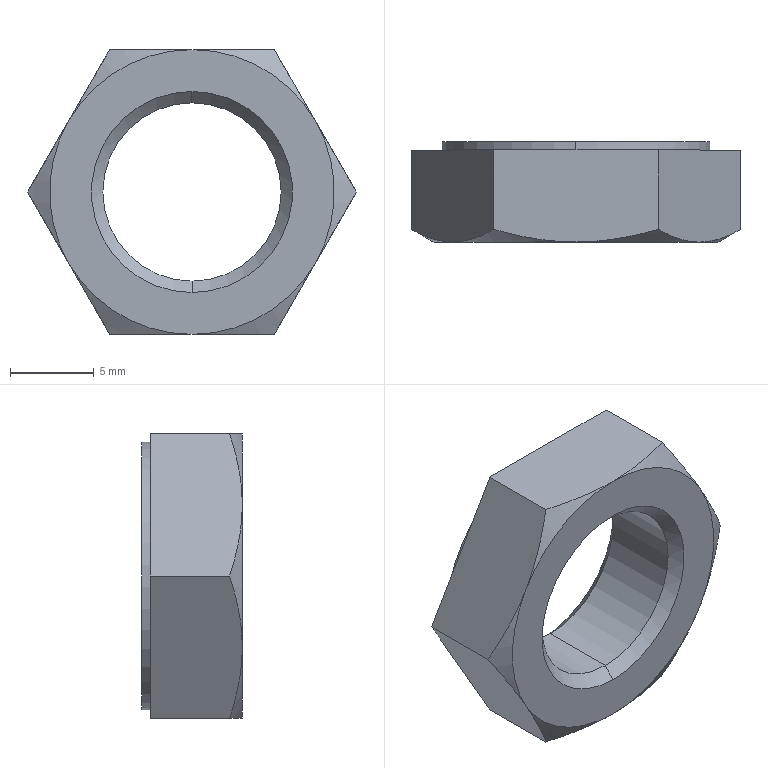Component | SolidWorks | MI-8x60-S-U-M-2(0)-1_MI8-M12x1_25 - Nut-1 | 1 solid | 23 faces | box 19.63 x 6 x 17 mm | volume 922 mm3 | cone 10 | plane 9 | cylinder 4 | commonest cylinder face diameters 10.647 x2 16 x2
build123d program:
from build123d import *

# Parameters (mm, degrees)
SKETCH2_W          = 34
SKETCH2_H          = 34
CUT_EXTRUDE1_DEPTH = 12


with BuildPart() as part:
    # Sketch1 → Revolve1 (revolve)
    with BuildSketch(Plane.XY, mode=Mode.PRIVATE) as revolve1_sk:
        Polygon((0, 0), (0, 8.5), (0.9815, 10.2), (5.5, 10.2), (5.5, 8), (6, 8), (6, 0), align=None)
    revolve(revolve1_sk.sketch.rotate(Axis((6, 0, 0), (-1, 0, 0)), 270), axis=Axis((6, 0, 0), (-1, 0, 0)))

    # Sketch2 → Cut-Extrude1 (cut)
    with BuildSketch(Plane(origin=(0, 0, 0), x_dir=(0, 0, -1), z_dir=(1, 0, 0))):
        Rectangle(SKETCH2_W, SKETCH2_H)
        Polygon((-8.5, 4.907), (-8.5, -4.907), (0, -9.815), (8.5, -4.907), (8.5, 4.907), (0, 9.815), align=None, mode=Mode.SUBTRACT)
    extrude(amount=CUT_EXTRUDE1_DEPTH, mode=Mode.SUBTRACT)

    # Sketch3 → Cut-Revolve1 (revolve, cut)
    with BuildSketch(Plane.XY, mode=Mode.PRIVATE) as cut_revolve1_sk:
        Polygon((0, 0), (0, 6), (0.6765, 5.324), (5.324, 5.324), (6, 6), (6, 0), align=None)
    revolve(cut_revolve1_sk.sketch.rotate(Axis((6, 0, 0), (-1, 0, 0)), 270), axis=Axis((6, 0, 0), (-1, 0, 0)), mode=Mode.SUBTRACT)


solid = part.part

# Placed as in the assembly
solid = solid.moved(Location((-44.181, -56.188, -311.979), (0, 0, 90)))
STEP:
#1=COLOUR_RGB('',0.7922,0.8196,0.9333);
#2=FILL_AREA_STYLE_COLOUR('',#1);
#3=FILL_AREA_STYLE('',(#2));
#4=SURFACE_STYLE_FILL_AREA(#3);
#5=SURFACE_SIDE_STYLE('',(#4));
#6=SURFACE_STYLE_USAGE(.BOTH.,#5);
#7=PRESENTATION_STYLE_ASSIGNMENT((#6));
#8=CARTESIAN_POINT('',(-1.739,-2.003,-12.073));
#9=VERTEX_POINT('',#8);
#10=CARTESIAN_POINT('',(-1.739,-2.003,-12.492));
#11=VERTEX_POINT('',#10);
#12=CARTESIAN_POINT('',(-1.739,-2.003,-12.283));
#13=DIRECTION('',(0.,-1.,0.));
#14=DIRECTION('',(0.,0.,-1.));
#15=AXIS2_PLACEMENT_3D('',#12,#13,#14);
#16=CIRCLE('',#15,0.2096);
#17=EDGE_CURVE('',#9,#11,#16,.T.);
#18=ORIENTED_EDGE('',*,*,#17,.T.);
#19=CARTESIAN_POINT('',(-1.739,-1.976,-12.519));
#20=VERTEX_POINT('',#19);
#21=CARTESIAN_POINT('',(-1.739,-1.976,-12.519));
#22=DIRECTION('',(0.,0.7071,-0.7071));
#23=VECTOR('',#22,39.37);
#24=LINE('',#21,#23);
#25=EDGE_CURVE('',#11,#20,#24,.T.);
#26=ORIENTED_EDGE('',*,*,#25,.T.);
#27=CARTESIAN_POINT('',(-1.739,-1.976,-12.046));
#28=VERTEX_POINT('',#27);
#29=CARTESIAN_POINT('',(-1.739,-1.976,-12.283));
#30=DIRECTION('',(0.,-1.,0.));
#31=DIRECTION('',(0.,0.,-1.));
#32=AXIS2_PLACEMENT_3D('',#29,#30,#31);
#33=CIRCLE('',#32,0.2362);
#34=EDGE_CURVE('',#28,#20,#33,.T.);
#35=ORIENTED_EDGE('',*,*,#34,.F.);
#36=CARTESIAN_POINT('',(-1.739,-1.976,-12.046));
#37=DIRECTION('',(-0.,0.7071,0.7071));
#38=VECTOR('',#37,39.37);
#39=LINE('',#36,#38);
#40=EDGE_CURVE('',#9,#28,#39,.T.);
#41=ORIENTED_EDGE('',*,*,#40,.F.);
#42=EDGE_LOOP('',(#18,#26,#35,#41));
#43=FACE_OUTER_BOUND('',#42,.T.);
#44=CARTESIAN_POINT('',(-1.739,-1.976,-12.283));
#45=DIRECTION('',(-0.,1.,-0.));
#46=DIRECTION('',(-0.,0.,1.));
#47=AXIS2_PLACEMENT_3D('',#44,#45,#46);
#48=CONICAL_SURFACE('',#47,0.2362,0.7854);
#49=ADVANCED_FACE('',(#43),#48,.F.);
#50=ORIENTED_EDGE('',*,*,#17,.F.);
#51=CARTESIAN_POINT('',(-1.739,-2.185,-12.073));
#52=VERTEX_POINT('',#51);
#53=CARTESIAN_POINT('',(-1.739,-1.976,-12.073));
#54=DIRECTION('',(0.,-1.,0.));
#55=VECTOR('',#54,39.37);
#56=LINE('',#53,#55);
#57=EDGE_CURVE('',#9,#52,#56,.T.);
#58=ORIENTED_EDGE('',*,*,#57,.T.);
#59=CARTESIAN_POINT('',(-1.739,-2.185,-12.492));
#60=VERTEX_POINT('',#59);
#61=CARTESIAN_POINT('',(-1.739,-2.185,-12.283));
#62=DIRECTION('',(0.,-1.,0.));
#63=DIRECTION('',(0.,0.,-1.));
#64=AXIS2_PLACEMENT_3D('',#61,#62,#63);
#65=CIRCLE('',#64,0.2096);
#66=EDGE_CURVE('',#52,#60,#65,.T.);
#67=ORIENTED_EDGE('',*,*,#66,.T.);
#68=CARTESIAN_POINT('',(-1.739,-1.976,-12.492));
#69=DIRECTION('',(0.,-1.,0.));
#70=VECTOR('',#69,39.37);
#71=LINE('',#68,#70);
#72=EDGE_CURVE('',#11,#60,#71,.T.);
#73=ORIENTED_EDGE('',*,*,#72,.F.);
#74=EDGE_LOOP('',(#50,#58,#67,#73));
#75=FACE_OUTER_BOUND('',#74,.T.);
#76=CARTESIAN_POINT('',(-1.739,-1.976,-12.283));
#77=DIRECTION('',(0.,-1.,0.));
#78=DIRECTION('',(0.,0.,-1.));
#79=AXIS2_PLACEMENT_3D('',#76,#77,#78);
#80=CYLINDRICAL_SURFACE('',#79,0.2096);
#81=ADVANCED_FACE('',(#75),#80,.F.);
#82=ORIENTED_EDGE('',*,*,#66,.F.);
#83=CARTESIAN_POINT('',(-1.739,-2.212,-12.046));
#84=VERTEX_POINT('',#83);
#85=CARTESIAN_POINT('',(-1.739,-2.185,-12.073));
#86=DIRECTION('',(-0.,-0.7071,0.7071));
#87=VECTOR('',#86,39.37);
#88=LINE('',#85,#87);
#89=EDGE_CURVE('',#52,#84,#88,.T.);
#90=ORIENTED_EDGE('',*,*,#89,.T.);
#91=CARTESIAN_POINT('',(-1.739,-2.212,-12.519));
#92=VERTEX_POINT('',#91);
#93=CARTESIAN_POINT('',(-1.739,-2.212,-12.283));
#94=DIRECTION('',(0.,-1.,0.));
#95=DIRECTION('',(0.,0.,-1.));
#96=AXIS2_PLACEMENT_3D('',#93,#94,#95);
#97=CIRCLE('',#96,0.2362);
#98=EDGE_CURVE('',#84,#92,#97,.T.);
#99=ORIENTED_EDGE('',*,*,#98,.T.);
#100=CARTESIAN_POINT('',(-1.739,-2.185,-12.492));
#101=DIRECTION('',(0.,-0.7071,-0.7071));
#102=VECTOR('',#101,39.37);
#103=LINE('',#100,#102);
#104=EDGE_CURVE('',#60,#92,#103,.T.);
#105=ORIENTED_EDGE('',*,*,#104,.F.);
#106=EDGE_LOOP('',(#82,#90,#99,#105));
#107=FACE_OUTER_BOUND('',#106,.T.);
#108=CARTESIAN_POINT('',(-1.739,-2.185,-12.283));
#109=DIRECTION('',(0.,-1.,0.));
#110=DIRECTION('',(0.,0.,-1.));
#111=AXIS2_PLACEMENT_3D('',#108,#109,#110);
#112=CONICAL_SURFACE('',#111,0.2096,0.7854);
#113=ADVANCED_FACE('',(#107),#112,.F.);
#114=CARTESIAN_POINT('',(-1.739,-1.976,-12.598));
#115=VERTEX_POINT('',#114);
#116=CARTESIAN_POINT('',(-1.739,-1.976,-11.968));
#117=VERTEX_POINT('',#116);
#118=CARTESIAN_POINT('',(-1.739,-1.976,-12.283));
#119=DIRECTION('',(0.,-1.,0.));
#120=DIRECTION('',(0.,0.,-1.));
#121=AXIS2_PLACEMENT_3D('',#118,#119,#120);
#122=CIRCLE('',#121,0.315);
#123=EDGE_CURVE('',#115,#117,#122,.T.);
#124=ORIENTED_EDGE('',*,*,#123,.T.);
#125=CARTESIAN_POINT('',(-1.739,-1.996,-11.968));
#126=VERTEX_POINT('',#125);
#127=CARTESIAN_POINT('',(-1.739,-1.976,-11.968));
#128=DIRECTION('',(0.,-1.,0.));
#129=VECTOR('',#128,39.37);
#130=LINE('',#127,#129);
#131=EDGE_CURVE('',#117,#126,#130,.T.);
#132=ORIENTED_EDGE('',*,*,#131,.T.);
#133=CARTESIAN_POINT('',(-1.739,-1.996,-12.598));
#134=VERTEX_POINT('',#133);
#135=CARTESIAN_POINT('',(-1.739,-1.996,-12.283));
#136=DIRECTION('',(0.,-1.,0.));
#137=DIRECTION('',(0.,0.,-1.));
#138=AXIS2_PLACEMENT_3D('',#135,#136,#137);
#139=CIRCLE('',#138,0.315);
#140=EDGE_CURVE('',#134,#126,#139,.T.);
#141=ORIENTED_EDGE('',*,*,#140,.F.);
#142=CARTESIAN_POINT('',(-1.739,-1.976,-12.598));
#143=DIRECTION('',(0.,-1.,0.));
#144=VECTOR('',#143,39.37);
#145=LINE('',#142,#144);
#146=EDGE_CURVE('',#115,#134,#145,.T.);
#147=ORIENTED_EDGE('',*,*,#146,.F.);
#148=EDGE_LOOP('',(#124,#132,#141,#147));
#149=FACE_OUTER_BOUND('',#148,.T.);
#150=CARTESIAN_POINT('',(-1.739,-1.976,-12.283));
#151=DIRECTION('',(0.,-1.,0.));
#152=DIRECTION('',(0.,0.,-1.));
#153=AXIS2_PLACEMENT_3D('',#150,#151,#152);
#154=CYLINDRICAL_SURFACE('',#153,0.315);
#155=ADVANCED_FACE('',(#149),#154,.T.);
#156=ORIENTED_EDGE('',*,*,#123,.F.);
#157=CARTESIAN_POINT('',(-1.739,-1.976,-12.283));
#158=DIRECTION('',(0.,-1.,0.));
#159=DIRECTION('',(0.,0.,-1.));
#160=AXIS2_PLACEMENT_3D('',#157,#158,#159);
#161=CIRCLE('',#160,0.315);
#162=EDGE_CURVE('',#117,#115,#161,.T.);
#163=ORIENTED_EDGE('',*,*,#162,.F.);
#164=EDGE_LOOP('',(#156,#163));
#165=FACE_OUTER_BOUND('',#164,.T.);
#166=ORIENTED_EDGE('',*,*,#34,.T.);
#167=CARTESIAN_POINT('',(-1.739,-1.976,-12.283));
#168=DIRECTION('',(0.,-1.,0.));
#169=DIRECTION('',(0.,0.,-1.));
#170=AXIS2_PLACEMENT_3D('',#167,#168,#169);
#171=CIRCLE('',#170,0.2362);
#172=EDGE_CURVE('',#20,#28,#171,.T.);
#173=ORIENTED_EDGE('',*,*,#172,.T.);
#174=EDGE_LOOP('',(#166,#173));
#175=FACE_BOUND('',#174,.T.);
#176=CARTESIAN_POINT('',(-1.424,-1.976,-12.283));
#177=DIRECTION('',(0.,-1.,0.));
#178=DIRECTION('',(0.,-0.,-1.));
#179=AXIS2_PLACEMENT_3D('',#176,#177,#178);
#180=PLANE('',#179);
#181=ADVANCED_FACE('',(#165,#175),#180,.F.);
#182=CARTESIAN_POINT('',(-1.739,-2.212,-12.617));
#183=VERTEX_POINT('',#182);
#184=CARTESIAN_POINT('',(-1.45,-2.212,-12.45));
#185=VERTEX_POINT('',#184);
#186=CARTESIAN_POINT('',(-1.739,-2.212,-12.283));
#187=DIRECTION('',(0.,-1.,0.));
#188=DIRECTION('',(0.,0.,-1.));
#189=AXIS2_PLACEMENT_3D('',#186,#187,#188);
#190=CIRCLE('',#189,0.3346);
#191=EDGE_CURVE('',#183,#185,#190,.T.);
#192=ORIENTED_EDGE('',*,*,#191,.T.);
#193=CARTESIAN_POINT('',(-1.45,-2.212,-12.115));
#194=VERTEX_POINT('',#193);
#195=CARTESIAN_POINT('',(-1.739,-2.212,-12.283));
#196=DIRECTION('',(0.,-1.,0.));
#197=DIRECTION('',(0.,0.,-1.));
#198=AXIS2_PLACEMENT_3D('',#195,#196,#197);
#199=CIRCLE('',#198,0.3346);
#200=EDGE_CURVE('',#185,#194,#199,.T.);
#201=ORIENTED_EDGE('',*,*,#200,.T.);
#202=CARTESIAN_POINT('',(-1.739,-2.212,-11.948));
#203=VERTEX_POINT('',#202);
#204=CARTESIAN_POINT('',(-1.739,-2.212,-12.283));
#205=DIRECTION('',(0.,-1.,0.));
#206=DIRECTION('',(0.,0.,-1.));
#207=AXIS2_PLACEMENT_3D('',#204,#205,#206);
#208=CIRCLE('',#207,0.3346);
#209=EDGE_CURVE('',#194,#203,#208,.T.);
#210=ORIENTED_EDGE('',*,*,#209,.T.);
#211=CARTESIAN_POINT('',(-2.029,-2.212,-12.115));
#212=VERTEX_POINT('',#211);
#213=CARTESIAN_POINT('',(-1.739,-2.212,-12.283));
#214=DIRECTION('',(0.,-1.,0.));
#215=DIRECTION('',(0.,0.,-1.));
#216=AXIS2_PLACEMENT_3D('',#213,#214,#215);
#217=CIRCLE('',#216,0.3346);
#218=EDGE_CURVE('',#203,#212,#217,.T.);
#219=ORIENTED_EDGE('',*,*,#218,.T.);
#220=CARTESIAN_POINT('',(-2.029,-2.212,-12.45));
#221=VERTEX_POINT('',#220);
#222=CARTESIAN_POINT('',(-1.739,-2.212,-12.283));
#223=DIRECTION('',(0.,-1.,0.));
#224=DIRECTION('',(0.,0.,-1.));
#225=AXIS2_PLACEMENT_3D('',#222,#223,#224);
#226=CIRCLE('',#225,0.3346);
#227=EDGE_CURVE('',#212,#221,#226,.T.);
#228=ORIENTED_EDGE('',*,*,#227,.T.);
#229=CARTESIAN_POINT('',(-1.739,-2.212,-12.283));
#230=DIRECTION('',(0.,-1.,0.));
#231=DIRECTION('',(0.,0.,-1.));
#232=AXIS2_PLACEMENT_3D('',#229,#230,#231);
#233=CIRCLE('',#232,0.3346);
#234=EDGE_CURVE('',#221,#183,#233,.T.);
#235=ORIENTED_EDGE('',*,*,#234,.T.);
#236=EDGE_LOOP('',(#192,#201,#210,#219,#228,#235));
#237=FACE_OUTER_BOUND('',#236,.T.);
#238=CARTESIAN_POINT('',(-1.739,-2.212,-12.283));
#239=DIRECTION('',(0.,-1.,0.));
#240=DIRECTION('',(0.,0.,-1.));
#241=AXIS2_PLACEMENT_3D('',#238,#239,#240);
#242=CIRCLE('',#241,0.2362);
#243=EDGE_CURVE('',#92,#84,#242,.T.);
#244=ORIENTED_EDGE('',*,*,#243,.F.);
#245=ORIENTED_EDGE('',*,*,#98,.F.);
#246=EDGE_LOOP('',(#244,#245));
#247=FACE_BOUND('',#246,.T.);
#248=CARTESIAN_POINT('',(-1.739,-2.212,-12.283));
#249=DIRECTION('',(-0.,1.,-0.));
#250=DIRECTION('',(-0.,0.,1.));
#251=AXIS2_PLACEMENT_3D('',#248,#249,#250);
#252=PLANE('',#251);
#253=ADVANCED_FACE('',(#237,#247),#252,.F.);
#254=CARTESIAN_POINT('',(-1.546,-1.996,-11.948));
#255=VERTEX_POINT('',#254);
#256=CARTESIAN_POINT('',(-1.353,-1.996,-12.283));
#257=VERTEX_POINT('',#256);
#258=CARTESIAN_POINT('',(-1.349,-1.996,-12.289));
#259=DIRECTION('',(0.5,0.,-0.866));
#260=VECTOR('',#259,39.37);
#261=LINE('',#258,#260);
#262=EDGE_CURVE('',#255,#257,#261,.T.);
#263=ORIENTED_EDGE('',*,*,#262,.T.);
#264=CARTESIAN_POINT('',(-1.546,-1.996,-12.617));
#265=VERTEX_POINT('',#264);
#266=CARTESIAN_POINT('',(-1.349,-1.996,-12.276));
#267=DIRECTION('',(-0.5,-0.,-0.866));
#268=VECTOR('',#267,39.37);
#269=LINE('',#266,#268);
#270=EDGE_CURVE('',#257,#265,#269,.T.);
#271=ORIENTED_EDGE('',*,*,#270,.T.);
#272=CARTESIAN_POINT('',(-1.933,-1.996,-12.617));
#273=VERTEX_POINT('',#272);
#274=CARTESIAN_POINT('',(-1.338,-1.996,-12.617));
#275=DIRECTION('',(-1.,-0.,-0.));
#276=VECTOR('',#275,39.37);
#277=LINE('',#274,#276);
#278=EDGE_CURVE('',#265,#273,#277,.T.);
#279=ORIENTED_EDGE('',*,*,#278,.T.);
#280=CARTESIAN_POINT('',(-2.126,-1.996,-12.283));
#281=VERTEX_POINT('',#280);
#282=CARTESIAN_POINT('',(-1.929,-1.996,-12.624));
#283=DIRECTION('',(-0.5,-0.,0.866));
#284=VECTOR('',#283,39.37);
#285=LINE('',#282,#284);
#286=EDGE_CURVE('',#273,#281,#285,.T.);
#287=ORIENTED_EDGE('',*,*,#286,.T.);
#288=CARTESIAN_POINT('',(-1.933,-1.996,-11.948));
#289=VERTEX_POINT('',#288);
#290=CARTESIAN_POINT('',(-1.929,-1.996,-11.941));
#291=DIRECTION('',(0.5,0.,0.866));
#292=VECTOR('',#291,39.37);
#293=LINE('',#290,#292);
#294=EDGE_CURVE('',#281,#289,#293,.T.);
#295=ORIENTED_EDGE('',*,*,#294,.T.);
#296=CARTESIAN_POINT('',(-1.338,-1.996,-11.948));
#297=DIRECTION('',(1.,0.,0.));
#298=VECTOR('',#297,39.37);
#299=LINE('',#296,#298);
#300=EDGE_CURVE('',#289,#255,#299,.T.);
#301=ORIENTED_EDGE('',*,*,#300,.T.);
#302=EDGE_LOOP('',(#263,#271,#279,#287,#295,#301));
#303=FACE_OUTER_BOUND('',#302,.T.);
#304=ORIENTED_EDGE('',*,*,#140,.T.);
#305=CARTESIAN_POINT('',(-1.739,-1.996,-12.283));
#306=DIRECTION('',(0.,-1.,0.));
#307=DIRECTION('',(0.,0.,-1.));
#308=AXIS2_PLACEMENT_3D('',#305,#306,#307);
#309=CIRCLE('',#308,0.315);
#310=EDGE_CURVE('',#126,#134,#309,.T.);
#311=ORIENTED_EDGE('',*,*,#310,.T.);
#312=EDGE_LOOP('',(#304,#311));
#313=FACE_BOUND('',#312,.T.);
#314=CARTESIAN_POINT('',(-1.338,-1.996,-12.283));
#315=DIRECTION('',(0.,-1.,0.));
#316=DIRECTION('',(0.,-0.,-1.));
#317=AXIS2_PLACEMENT_3D('',#314,#315,#316);
#318=PLANE('',#317);
#319=ADVANCED_FACE('',(#303,#313),#318,.F.);
#320=ORIENTED_EDGE('',*,*,#131,.F.);
#321=ORIENTED_EDGE('',*,*,#162,.T.);
#322=ORIENTED_EDGE('',*,*,#146,.T.);
#323=ORIENTED_EDGE('',*,*,#310,.F.);
#324=EDGE_LOOP('',(#320,#321,#322,#323));
#325=FACE_OUTER_BOUND('',#324,.T.);
#326=CARTESIAN_POINT('',(-1.739,-1.976,-12.283));
#327=DIRECTION('',(0.,-1.,0.));
#328=DIRECTION('',(0.,0.,-1.));
#329=AXIS2_PLACEMENT_3D('',#326,#327,#328);
#330=CYLINDRICAL_SURFACE('',#329,0.315);
#331=ADVANCED_FACE('',(#325),#330,.T.);
#332=CARTESIAN_POINT('',(-1.546,-2.182,-12.617));
#333=VERTEX_POINT('',#332);
#334=CARTESIAN_POINT('',(-1.546,-1.74,-12.617));
#335=DIRECTION('',(0.,-1.,0.));
#336=VECTOR('',#335,39.37);
#337=LINE('',#334,#336);
#338=EDGE_CURVE('',#265,#333,#337,.T.);
#339=ORIENTED_EDGE('',*,*,#338,.F.);
#340=ORIENTED_EDGE('',*,*,#270,.F.);
#341=CARTESIAN_POINT('',(-1.353,-2.182,-12.283));
#342=VERTEX_POINT('',#341);
#343=CARTESIAN_POINT('',(-1.353,-1.74,-12.283));
#344=DIRECTION('',(0.,-1.,0.));
#345=VECTOR('',#344,39.37);
#346=LINE('',#343,#345);
#347=EDGE_CURVE('',#257,#342,#346,.T.);
#348=ORIENTED_EDGE('',*,*,#347,.T.);
#349=CARTESIAN_POINT('',(-1.45,-2.212,-12.45));
#350=CARTESIAN_POINT('',(-1.441,-2.212,-12.436));
#351=CARTESIAN_POINT('',(-1.433,-2.211,-12.421));
#352=CARTESIAN_POINT('',(-1.417,-2.209,-12.393));
#353=CARTESIAN_POINT('',(-1.409,-2.207,-12.379));
#354=CARTESIAN_POINT('',(-1.385,-2.199,-12.337));
#355=CARTESIAN_POINT('',(-1.369,-2.191,-12.31));
#356=CARTESIAN_POINT('',(-1.353,-2.182,-12.283));
#357=B_SPLINE_CURVE_WITH_KNOTS('',3,(#349,#350,#351,#352,#353,#354,#355,#356),.UNSPECIFIED.,.F.,.F.,(4,2,2,4),(0.004966,0.006203,0.007439,0.009913),.UNSPECIFIED.);
#358=EDGE_CURVE('',#185,#342,#357,.T.);
#359=ORIENTED_EDGE('',*,*,#358,.F.);
#360=CARTESIAN_POINT('',(-1.546,-2.182,-12.617));
#361=CARTESIAN_POINT('',(-1.53,-2.191,-12.59));
#362=CARTESIAN_POINT('',(-1.514,-2.199,-12.562));
#363=CARTESIAN_POINT('',(-1.482,-2.209,-12.507));
#364=CARTESIAN_POINT('',(-1.466,-2.212,-12.478));
#365=CARTESIAN_POINT('',(-1.45,-2.212,-12.45));
#366=B_SPLINE_CURVE_WITH_KNOTS('',3,(#360,#361,#362,#363,#364,#365),.UNSPECIFIED.,.F.,.F.,(4,2,4),(0.00000024,0.002483,0.004966),.UNSPECIFIED.);
#367=EDGE_CURVE('',#333,#185,#366,.T.);
#368=ORIENTED_EDGE('',*,*,#367,.F.);
#369=EDGE_LOOP('',(#339,#340,#348,#359,#368));
#370=FACE_OUTER_BOUND('',#369,.T.);
#371=CARTESIAN_POINT('',(-1.353,-1.74,-12.283));
#372=DIRECTION('',(-0.866,-0.,0.5));
#373=DIRECTION('',(0.5,0.,0.866));
#374=AXIS2_PLACEMENT_3D('',#371,#372,#373);
#375=PLANE('',#374);
#376=ADVANCED_FACE('',(#370),#375,.F.);
#377=CARTESIAN_POINT('',(-1.933,-2.182,-12.617));
#378=VERTEX_POINT('',#377);
#379=CARTESIAN_POINT('',(-1.933,-1.74,-12.617));
#380=DIRECTION('',(0.,-1.,0.));
#381=VECTOR('',#380,39.37);
#382=LINE('',#379,#381);
#383=EDGE_CURVE('',#273,#378,#382,.T.);
#384=ORIENTED_EDGE('',*,*,#383,.F.);
#385=ORIENTED_EDGE('',*,*,#278,.F.);
#386=ORIENTED_EDGE('',*,*,#338,.T.);
#387=CARTESIAN_POINT('',(-1.739,-2.212,-12.617));
#388=CARTESIAN_POINT('',(-1.707,-2.212,-12.617));
#389=CARTESIAN_POINT('',(-1.674,-2.209,-12.617));
#390=CARTESIAN_POINT('',(-1.609,-2.199,-12.617));
#391=CARTESIAN_POINT('',(-1.577,-2.191,-12.617));
#392=CARTESIAN_POINT('',(-1.546,-2.182,-12.617));
#393=B_SPLINE_CURVE_WITH_KNOTS('',3,(#387,#388,#389,#390,#391,#392),.UNSPECIFIED.,.F.,.F.,(4,2,4),(0.01375,0.01624,0.01872),.UNSPECIFIED.);
#394=EDGE_CURVE('',#183,#333,#393,.T.);
#395=ORIENTED_EDGE('',*,*,#394,.F.);
#396=CARTESIAN_POINT('',(-1.933,-2.182,-12.617));
#397=CARTESIAN_POINT('',(-1.901,-2.191,-12.617));
#398=CARTESIAN_POINT('',(-1.869,-2.199,-12.617));
#399=CARTESIAN_POINT('',(-1.804,-2.209,-12.617));
#400=CARTESIAN_POINT('',(-1.772,-2.212,-12.617));
#401=CARTESIAN_POINT('',(-1.739,-2.212,-12.617));
#402=B_SPLINE_CURVE_WITH_KNOTS('',3,(#396,#397,#398,#399,#400,#401),.UNSPECIFIED.,.F.,.F.,(4,2,4),(0.00879,0.01127,0.01375),.UNSPECIFIED.);
#403=EDGE_CURVE('',#378,#183,#402,.T.);
#404=ORIENTED_EDGE('',*,*,#403,.F.);
#405=EDGE_LOOP('',(#384,#385,#386,#395,#404));
#406=FACE_OUTER_BOUND('',#405,.T.);
#407=CARTESIAN_POINT('',(-1.546,-1.74,-12.617));
#408=DIRECTION('',(-0.,0.,1.));
#409=DIRECTION('',(0.,-1.,0.));
#410=AXIS2_PLACEMENT_3D('',#407,#408,#409);
#411=PLANE('',#410);
#412=ADVANCED_FACE('',(#406),#411,.F.);
#413=CARTESIAN_POINT('',(-2.126,-2.182,-12.283));
#414=VERTEX_POINT('',#413);
#415=CARTESIAN_POINT('',(-2.126,-1.74,-12.283));
#416=DIRECTION('',(0.,-1.,0.));
#417=VECTOR('',#416,39.37);
#418=LINE('',#415,#417);
#419=EDGE_CURVE('',#281,#414,#418,.T.);
#420=ORIENTED_EDGE('',*,*,#419,.F.);
#421=ORIENTED_EDGE('',*,*,#286,.F.);
#422=ORIENTED_EDGE('',*,*,#383,.T.);
#423=CARTESIAN_POINT('',(-2.029,-2.212,-12.45));
#424=CARTESIAN_POINT('',(-2.021,-2.212,-12.464));
#425=CARTESIAN_POINT('',(-2.013,-2.211,-12.478));
#426=CARTESIAN_POINT('',(-1.996,-2.209,-12.507));
#427=CARTESIAN_POINT('',(-1.988,-2.207,-12.521));
#428=CARTESIAN_POINT('',(-1.964,-2.199,-12.562));
#429=CARTESIAN_POINT('',(-1.948,-2.191,-12.59));
#430=CARTESIAN_POINT('',(-1.933,-2.182,-12.617));
#431=B_SPLINE_CURVE_WITH_KNOTS('',3,(#423,#424,#425,#426,#427,#428,#429,#430),.UNSPECIFIED.,.F.,.F.,(4,2,2,4),(0.004966,0.006203,0.007439,0.009913),.UNSPECIFIED.);
#432=EDGE_CURVE('',#221,#378,#431,.T.);
#433=ORIENTED_EDGE('',*,*,#432,.F.);
#434=CARTESIAN_POINT('',(-2.126,-2.182,-12.283));
#435=CARTESIAN_POINT('',(-2.11,-2.191,-12.31));
#436=CARTESIAN_POINT('',(-2.094,-2.199,-12.338));
#437=CARTESIAN_POINT('',(-2.062,-2.209,-12.393));
#438=CARTESIAN_POINT('',(-2.046,-2.212,-12.421));
#439=CARTESIAN_POINT('',(-2.029,-2.212,-12.45));
#440=B_SPLINE_CURVE_WITH_KNOTS('',3,(#434,#435,#436,#437,#438,#439),.UNSPECIFIED.,.F.,.F.,(4,2,4),(0.00000024,0.002483,0.004966),.UNSPECIFIED.);
#441=EDGE_CURVE('',#414,#221,#440,.T.);
#442=ORIENTED_EDGE('',*,*,#441,.F.);
#443=EDGE_LOOP('',(#420,#421,#422,#433,#442));
#444=FACE_OUTER_BOUND('',#443,.T.);
#445=CARTESIAN_POINT('',(-1.933,-1.74,-12.617));
#446=DIRECTION('',(0.866,0.,0.5));
#447=DIRECTION('',(0.5,0.,-0.866));
#448=AXIS2_PLACEMENT_3D('',#445,#446,#447);
#449=PLANE('',#448);
#450=ADVANCED_FACE('',(#444),#449,.F.);
#451=CARTESIAN_POINT('',(-1.933,-2.182,-11.948));
#452=VERTEX_POINT('',#451);
#453=CARTESIAN_POINT('',(-1.933,-1.74,-11.948));
#454=DIRECTION('',(0.,-1.,0.));
#455=VECTOR('',#454,39.37);
#456=LINE('',#453,#455);
#457=EDGE_CURVE('',#289,#452,#456,.T.);
#458=ORIENTED_EDGE('',*,*,#457,.F.);
#459=ORIENTED_EDGE('',*,*,#294,.F.);
#460=ORIENTED_EDGE('',*,*,#419,.T.);
#461=CARTESIAN_POINT('',(-2.029,-2.212,-12.115));
#462=CARTESIAN_POINT('',(-2.037,-2.212,-12.13));
#463=CARTESIAN_POINT('',(-2.046,-2.211,-12.144));
#464=CARTESIAN_POINT('',(-2.062,-2.209,-12.172));
#465=CARTESIAN_POINT('',(-2.07,-2.207,-12.186));
#466=CARTESIAN_POINT('',(-2.094,-2.199,-12.228));
#467=CARTESIAN_POINT('',(-2.11,-2.191,-12.255));
#468=CARTESIAN_POINT('',(-2.126,-2.182,-12.283));
#469=B_SPLINE_CURVE_WITH_KNOTS('',3,(#461,#462,#463,#464,#465,#466,#467,#468),.UNSPECIFIED.,.F.,.F.,(4,2,2,4),(0.004966,0.006203,0.007439,0.009913),.UNSPECIFIED.);
#470=EDGE_CURVE('',#212,#414,#469,.T.);
#471=ORIENTED_EDGE('',*,*,#470,.F.);
#472=CARTESIAN_POINT('',(-1.933,-2.182,-11.948));
#473=CARTESIAN_POINT('',(-1.948,-2.191,-11.975));
#474=CARTESIAN_POINT('',(-1.964,-2.199,-12.003));
#475=CARTESIAN_POINT('',(-1.996,-2.209,-12.059));
#476=CARTESIAN_POINT('',(-2.013,-2.212,-12.087));
#477=CARTESIAN_POINT('',(-2.029,-2.212,-12.115));
#478=B_SPLINE_CURVE_WITH_KNOTS('',3,(#472,#473,#474,#475,#476,#477),.UNSPECIFIED.,.F.,.F.,(4,2,4),(0.00000024,0.002483,0.004966),.UNSPECIFIED.);
#479=EDGE_CURVE('',#452,#212,#478,.T.);
#480=ORIENTED_EDGE('',*,*,#479,.F.);
#481=EDGE_LOOP('',(#458,#459,#460,#471,#480));
#482=FACE_OUTER_BOUND('',#481,.T.);
#483=CARTESIAN_POINT('',(-2.126,-1.74,-12.283));
#484=DIRECTION('',(0.866,0.,-0.5));
#485=DIRECTION('',(-0.5,-0.,-0.866));
#486=AXIS2_PLACEMENT_3D('',#483,#484,#485);
#487=PLANE('',#486);
#488=ADVANCED_FACE('',(#482),#487,.F.);
#489=CARTESIAN_POINT('',(-1.546,-2.182,-11.948));
#490=VERTEX_POINT('',#489);
#491=CARTESIAN_POINT('',(-1.546,-1.74,-11.948));
#492=DIRECTION('',(0.,-1.,0.));
#493=VECTOR('',#492,39.37);
#494=LINE('',#491,#493);
#495=EDGE_CURVE('',#255,#490,#494,.T.);
#496=ORIENTED_EDGE('',*,*,#495,.F.);
#497=ORIENTED_EDGE('',*,*,#300,.F.);
#498=ORIENTED_EDGE('',*,*,#457,.T.);
#499=CARTESIAN_POINT('',(-1.739,-2.212,-11.948));
#500=CARTESIAN_POINT('',(-1.772,-2.212,-11.948));
#501=CARTESIAN_POINT('',(-1.804,-2.209,-11.948));
#502=CARTESIAN_POINT('',(-1.869,-2.199,-11.948));
#503=CARTESIAN_POINT('',(-1.901,-2.191,-11.948));
#504=CARTESIAN_POINT('',(-1.933,-2.182,-11.948));
#505=B_SPLINE_CURVE_WITH_KNOTS('',3,(#499,#500,#501,#502,#503,#504),.UNSPECIFIED.,.F.,.F.,(4,2,4),(0.02652,0.029,0.03149),.UNSPECIFIED.);
#506=EDGE_CURVE('',#203,#452,#505,.T.);
#507=ORIENTED_EDGE('',*,*,#506,.F.);
#508=CARTESIAN_POINT('',(-1.546,-2.182,-11.948));
#509=CARTESIAN_POINT('',(-1.577,-2.191,-11.948));
#510=CARTESIAN_POINT('',(-1.609,-2.199,-11.948));
#511=CARTESIAN_POINT('',(-1.674,-2.209,-11.948));
#512=CARTESIAN_POINT('',(-1.707,-2.212,-11.948));
#513=CARTESIAN_POINT('',(-1.739,-2.212,-11.948));
#514=B_SPLINE_CURVE_WITH_KNOTS('',3,(#508,#509,#510,#511,#512,#513),.UNSPECIFIED.,.F.,.F.,(4,2,4),(0.02154,0.02403,0.02652),.UNSPECIFIED.);
#515=EDGE_CURVE('',#490,#203,#514,.T.);
#516=ORIENTED_EDGE('',*,*,#515,.F.);
#517=EDGE_LOOP('',(#496,#497,#498,#507,#516));
#518=FACE_OUTER_BOUND('',#517,.T.);
#519=CARTESIAN_POINT('',(-1.933,-1.74,-11.948));
#520=DIRECTION('',(0.,-0.,-1.));
#521=DIRECTION('',(-0.,1.,-0.));
#522=AXIS2_PLACEMENT_3D('',#519,#520,#521);
#523=PLANE('',#522);
#524=ADVANCED_FACE('',(#518),#523,.F.);
#525=ORIENTED_EDGE('',*,*,#347,.F.);
#526=ORIENTED_EDGE('',*,*,#262,.F.);
#527=ORIENTED_EDGE('',*,*,#495,.T.);
#528=CARTESIAN_POINT('',(-1.45,-2.212,-12.115));
#529=CARTESIAN_POINT('',(-1.458,-2.212,-12.101));
#530=CARTESIAN_POINT('',(-1.466,-2.211,-12.087));
#531=CARTESIAN_POINT('',(-1.482,-2.209,-12.059));
#532=CARTESIAN_POINT('',(-1.49,-2.207,-12.045));
#533=CARTESIAN_POINT('',(-1.515,-2.199,-12.003));
#534=CARTESIAN_POINT('',(-1.53,-2.191,-11.975));
#535=CARTESIAN_POINT('',(-1.546,-2.182,-11.948));
#536=B_SPLINE_CURVE_WITH_KNOTS('',3,(#528,#529,#530,#531,#532,#533,#534,#535),.UNSPECIFIED.,.F.,.F.,(4,2,2,4),(0.004966,0.006203,0.007439,0.009913),.UNSPECIFIED.);
#537=EDGE_CURVE('',#194,#490,#536,.T.);
#538=ORIENTED_EDGE('',*,*,#537,.F.);
#539=CARTESIAN_POINT('',(-1.353,-2.182,-12.283));
#540=CARTESIAN_POINT('',(-1.369,-2.191,-12.255));
#541=CARTESIAN_POINT('',(-1.385,-2.199,-12.228));
#542=CARTESIAN_POINT('',(-1.417,-2.209,-12.172));
#543=CARTESIAN_POINT('',(-1.433,-2.212,-12.144));
#544=CARTESIAN_POINT('',(-1.45,-2.212,-12.115));
#545=B_SPLINE_CURVE_WITH_KNOTS('',3,(#539,#540,#541,#542,#543,#544),.UNSPECIFIED.,.F.,.F.,(4,2,4),(0.00000024,0.002483,0.004966),.UNSPECIFIED.);
#546=EDGE_CURVE('',#342,#194,#545,.T.);
#547=ORIENTED_EDGE('',*,*,#546,.F.);
#548=EDGE_LOOP('',(#525,#526,#527,#538,#547));
#549=FACE_OUTER_BOUND('',#548,.T.);
#550=CARTESIAN_POINT('',(-1.546,-1.74,-11.948));
#551=DIRECTION('',(-0.866,-0.,-0.5));
#552=DIRECTION('',(-0.5,-0.,0.866));
#553=AXIS2_PLACEMENT_3D('',#550,#551,#552);
#554=PLANE('',#553);
#555=ADVANCED_FACE('',(#549),#554,.F.);
#556=ORIENTED_EDGE('',*,*,#234,.F.);
#557=ORIENTED_EDGE('',*,*,#432,.T.);
#558=ORIENTED_EDGE('',*,*,#403,.T.);
#559=EDGE_LOOP('',(#556,#557,#558));
#560=FACE_OUTER_BOUND('',#559,.T.);
#561=CARTESIAN_POINT('',(-1.739,-2.173,-12.283));
#562=DIRECTION('',(-0.,1.,-0.));
#563=DIRECTION('',(-0.,0.,1.));
#564=AXIS2_PLACEMENT_3D('',#561,#562,#563);
#565=CONICAL_SURFACE('',#564,0.4016,1.047);
#566=ADVANCED_FACE('',(#560),#565,.T.);
#567=ORIENTED_EDGE('',*,*,#470,.T.);
#568=ORIENTED_EDGE('',*,*,#441,.T.);
#569=ORIENTED_EDGE('',*,*,#227,.F.);
#570=EDGE_LOOP('',(#567,#568,#569));
#571=FACE_OUTER_BOUND('',#570,.T.);
#572=CARTESIAN_POINT('',(-1.739,-2.173,-12.283));
#573=DIRECTION('',(-0.,1.,-0.));
#574=DIRECTION('',(-0.,0.,1.));
#575=AXIS2_PLACEMENT_3D('',#572,#573,#574);
#576=CONICAL_SURFACE('',#575,0.4016,1.047);
#577=ADVANCED_FACE('',(#571),#576,.T.);
#578=ORIENTED_EDGE('',*,*,#506,.T.);
#579=ORIENTED_EDGE('',*,*,#479,.T.);
#580=ORIENTED_EDGE('',*,*,#218,.F.);
#581=EDGE_LOOP('',(#578,#579,#580));
#582=FACE_OUTER_BOUND('',#581,.T.);
#583=CARTESIAN_POINT('',(-1.739,-2.173,-12.283));
#584=DIRECTION('',(-0.,1.,-0.));
#585=DIRECTION('',(-0.,0.,1.));
#586=AXIS2_PLACEMENT_3D('',#583,#584,#585);
#587=CONICAL_SURFACE('',#586,0.4016,1.047);
#588=ADVANCED_FACE('',(#582),#587,.T.);
#589=ORIENTED_EDGE('',*,*,#200,.F.);
#590=ORIENTED_EDGE('',*,*,#358,.T.);
#591=ORIENTED_EDGE('',*,*,#546,.T.);
#592=EDGE_LOOP('',(#589,#590,#591));
#593=FACE_OUTER_BOUND('',#592,.T.);
#594=CARTESIAN_POINT('',(-1.739,-2.173,-12.283));
#595=DIRECTION('',(-0.,1.,-0.));
#596=DIRECTION('',(-0.,0.,1.));
#597=AXIS2_PLACEMENT_3D('',#594,#595,#596);
#598=CONICAL_SURFACE('',#597,0.4016,1.047);
#599=ADVANCED_FACE('',(#593),#598,.T.);
#600=ORIENTED_EDGE('',*,*,#191,.F.);
#601=ORIENTED_EDGE('',*,*,#394,.T.);
#602=ORIENTED_EDGE('',*,*,#367,.T.);
#603=EDGE_LOOP('',(#600,#601,#602));
#604=FACE_OUTER_BOUND('',#603,.T.);
#605=CARTESIAN_POINT('',(-1.739,-2.173,-12.283));
#606=DIRECTION('',(-0.,1.,-0.));
#607=DIRECTION('',(-0.,0.,1.));
#608=AXIS2_PLACEMENT_3D('',#605,#606,#607);
#609=CONICAL_SURFACE('',#608,0.4016,1.047);
#610=ADVANCED_FACE('',(#604),#609,.T.);
#611=ORIENTED_EDGE('',*,*,#537,.T.);
#612=ORIENTED_EDGE('',*,*,#515,.T.);
#613=ORIENTED_EDGE('',*,*,#209,.F.);
#614=EDGE_LOOP('',(#611,#612,#613));
#615=FACE_OUTER_BOUND('',#614,.T.);
#616=CARTESIAN_POINT('',(-1.739,-2.173,-12.283));
#617=DIRECTION('',(-0.,1.,-0.));
#618=DIRECTION('',(-0.,0.,1.));
#619=AXIS2_PLACEMENT_3D('',#616,#617,#618);
#620=CONICAL_SURFACE('',#619,0.4016,1.047);
#621=ADVANCED_FACE('',(#615),#620,.T.);
#622=ORIENTED_EDGE('',*,*,#89,.F.);
#623=CARTESIAN_POINT('',(-1.739,-2.185,-12.283));
#624=DIRECTION('',(0.,-1.,0.));
#625=DIRECTION('',(0.,0.,-1.));
#626=AXIS2_PLACEMENT_3D('',#623,#624,#625);
#627=CIRCLE('',#626,0.2096);
#628=EDGE_CURVE('',#60,#52,#627,.T.);
#629=ORIENTED_EDGE('',*,*,#628,.F.);
#630=ORIENTED_EDGE('',*,*,#104,.T.);
#631=ORIENTED_EDGE('',*,*,#243,.T.);
#632=EDGE_LOOP('',(#622,#629,#630,#631));
#633=FACE_OUTER_BOUND('',#632,.T.);
#634=CARTESIAN_POINT('',(-1.739,-2.185,-12.283));
#635=DIRECTION('',(0.,-1.,0.));
#636=DIRECTION('',(0.,0.,-1.));
#637=AXIS2_PLACEMENT_3D('',#634,#635,#636);
#638=CONICAL_SURFACE('',#637,0.2096,0.7854);
#639=ADVANCED_FACE('',(#633),#638,.F.);
#640=ORIENTED_EDGE('',*,*,#57,.F.);
#641=CARTESIAN_POINT('',(-1.739,-2.003,-12.283));
#642=DIRECTION('',(0.,-1.,0.));
#643=DIRECTION('',(0.,0.,-1.));
#644=AXIS2_PLACEMENT_3D('',#641,#642,#643);
#645=CIRCLE('',#644,0.2096);
#646=EDGE_CURVE('',#11,#9,#645,.T.);
#647=ORIENTED_EDGE('',*,*,#646,.F.);
#648=ORIENTED_EDGE('',*,*,#72,.T.);
#649=ORIENTED_EDGE('',*,*,#628,.T.);
#650=EDGE_LOOP('',(#640,#647,#648,#649));
#651=FACE_OUTER_BOUND('',#650,.T.);
#652=CARTESIAN_POINT('',(-1.739,-1.976,-12.283));
#653=DIRECTION('',(0.,-1.,0.));
#654=DIRECTION('',(0.,0.,-1.));
#655=AXIS2_PLACEMENT_3D('',#652,#653,#654);
#656=CYLINDRICAL_SURFACE('',#655,0.2096);
#657=ADVANCED_FACE('',(#651),#656,.F.);
#658=ORIENTED_EDGE('',*,*,#25,.F.);
#659=ORIENTED_EDGE('',*,*,#646,.T.);
#660=ORIENTED_EDGE('',*,*,#40,.T.);
#661=ORIENTED_EDGE('',*,*,#172,.F.);
#662=EDGE_LOOP('',(#658,#659,#660,#661));
#663=FACE_OUTER_BOUND('',#662,.T.);
#664=CARTESIAN_POINT('',(-1.739,-1.976,-12.283));
#665=DIRECTION('',(-0.,1.,-0.));
#666=DIRECTION('',(-0.,0.,1.));
#667=AXIS2_PLACEMENT_3D('',#664,#665,#666);
#668=CONICAL_SURFACE('',#667,0.2362,0.7854);
#669=ADVANCED_FACE('',(#663),#668,.F.);
#670=CLOSED_SHELL('',(#49,#81,#113,#155,#181,#253,#319,#331,#376,#412,#450,#488,#524,#555,#566,#577,#588,#599,#610,#621,#639,#657,#669));
#671=MANIFOLD_SOLID_BREP('',#670);
#672=STYLED_ITEM('',(#7),#671);
#673=(LENGTH_UNIT()NAMED_UNIT(*)SI_UNIT($,.METRE.));
#674=LENGTH_MEASURE_WITH_UNIT(LENGTH_MEASURE(0.0254),#673);
#675=DIMENSIONAL_EXPONENTS(1.,0.,0.,0.,0.,0.,0.);
#676=(CONVERSION_BASED_UNIT('',#674)LENGTH_UNIT()NAMED_UNIT(#675));
#677=UNCERTAINTY_MEASURE_WITH_UNIT(LENGTH_MEASURE(0.00001),#676,'','');
#678=(NAMED_UNIT(*)PLANE_ANGLE_UNIT()SI_UNIT($,.RADIAN.));
#679=(NAMED_UNIT(*)SI_UNIT($,.STERADIAN.)SOLID_ANGLE_UNIT());
#680=(GEOMETRIC_REPRESENTATION_CONTEXT(3)GLOBAL_UNCERTAINTY_ASSIGNED_CONTEXT((#677))GLOBAL_UNIT_ASSIGNED_CONTEXT((#676,#678,#679))REPRESENTATION_CONTEXT('',''));
#681=MECHANICAL_DESIGN_GEOMETRIC_PRESENTATION_REPRESENTATION('',(#672),#680);
#682=PRESENTATION_LAYER_ASSIGNMENT('','',(#672));
#683=CARTESIAN_POINT('',(0.,0.,0.));
#684=DIRECTION('',(0.,0.,1.));
#685=DIRECTION('',(1.,0.,0.));
#686=AXIS2_PLACEMENT_3D('',#683,#684,#685);
#687=(LENGTH_UNIT()NAMED_UNIT(*)SI_UNIT($,.METRE.));
#688=LENGTH_MEASURE_WITH_UNIT(LENGTH_MEASURE(0.0254),#687);
#689=DIMENSIONAL_EXPONENTS(1.,0.,0.,0.,0.,0.,0.);
#690=(CONVERSION_BASED_UNIT('',#688)LENGTH_UNIT()NAMED_UNIT(#689));
#691=UNCERTAINTY_MEASURE_WITH_UNIT(LENGTH_MEASURE(0.00001),#690,'','');
#692=(NAMED_UNIT(*)PLANE_ANGLE_UNIT()SI_UNIT($,.RADIAN.));
#693=(NAMED_UNIT(*)SI_UNIT($,.STERADIAN.)SOLID_ANGLE_UNIT());
#694=(GEOMETRIC_REPRESENTATION_CONTEXT(3)GLOBAL_UNCERTAINTY_ASSIGNED_CONTEXT((#691))GLOBAL_UNIT_ASSIGNED_CONTEXT((#690,#692,#693))REPRESENTATION_CONTEXT('',''));
#695=ADVANCED_BREP_SHAPE_REPRESENTATION('',(#671,#686),#694);